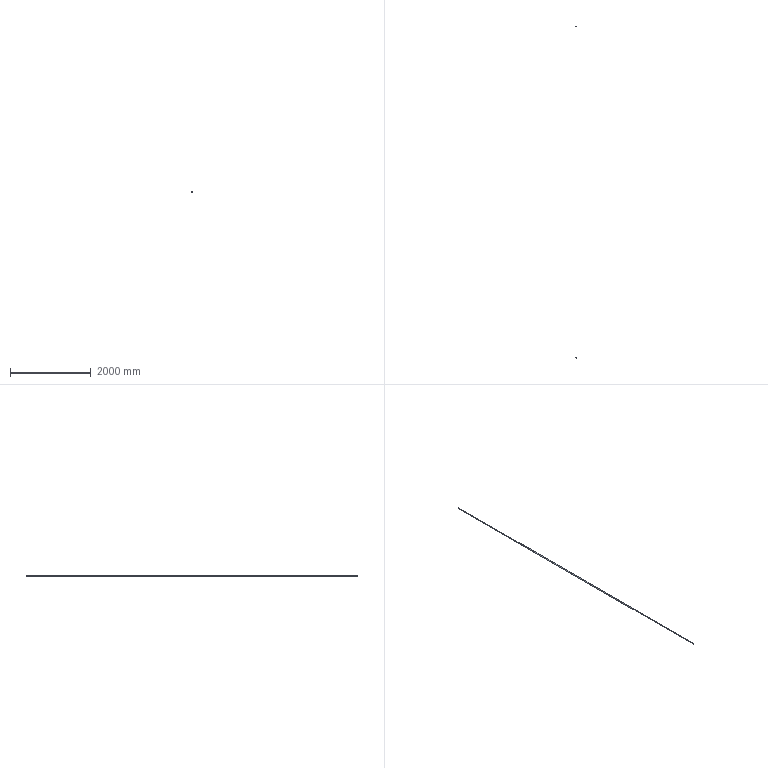Component | NX | 44 | 1 solid | 4 faces | volume 929660 mm3 | cylinder 2 | plane 2 | commonest cylinder face diameters 20 x1 16 x1